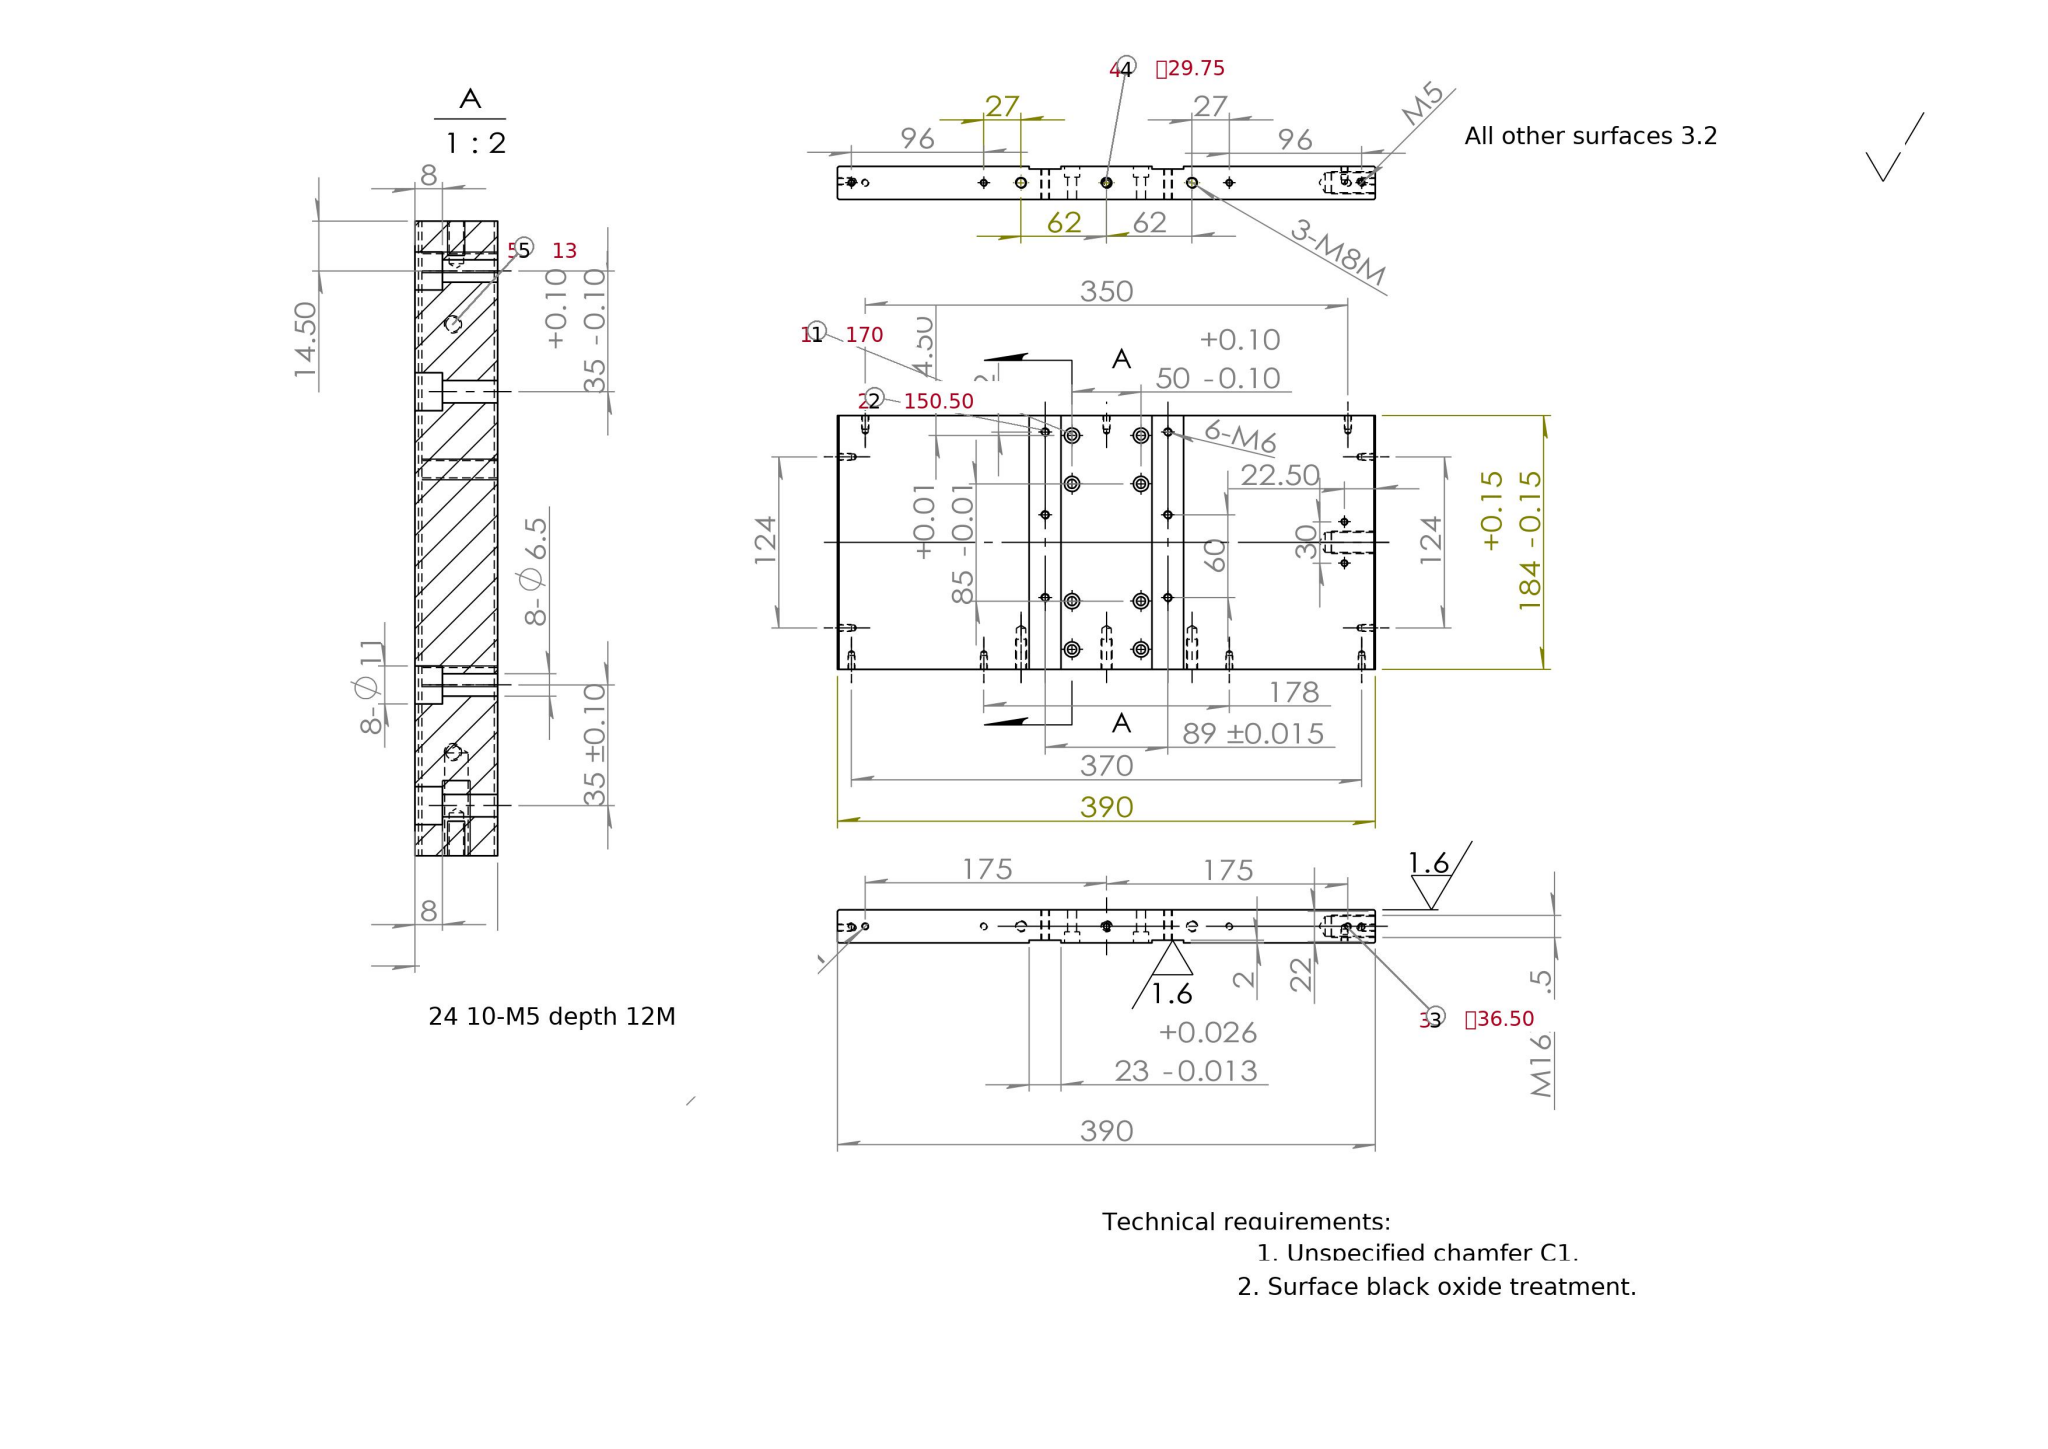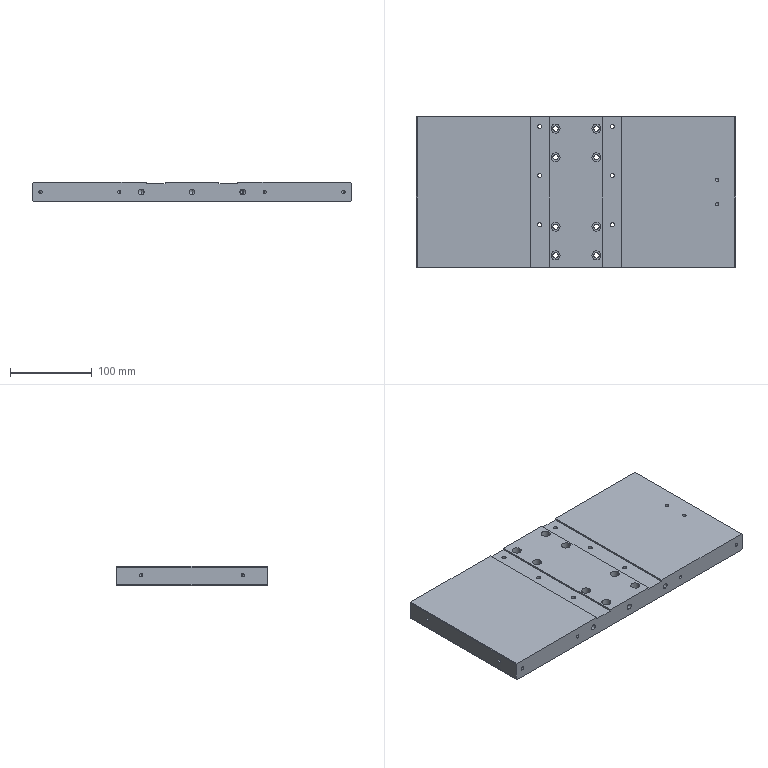Part | SolidWorks | mm | 1 solid | 138 faces | box 390 x 184 x 24 mm | volume 1680131 mm3 | cylinder 78 | cone 34 | plane 26 | commonest cylinder face diameters 4.2 x26 11 x16 6.5 x16 5 x12 6.8 x6 14.5 x2
build123d program:
from build123d import *

# Parameters (mm, degrees)
SKETCH1_W                            = 390
SKETCH1_H                            = 184
EXTRUDE1_DEPTH                       = 24
SKETCH2_R                            = 3.25
EXTRUDE2_DEPTH                       = 24
SKETCH3_R                            = 5.5
EXTRUDE3_DEPTH                       = 8
M5_TAPPED_HOLE2_AT_2_COUNT           = 2
M5_TAPPED_HOLE2_AT_2_PITCH           = 27.073
LPATTERN2_COUNT                      = 3
LPATTERN2_PITCH                      = 175
M5_TAPPED_HOLE5_D                    = 4.2
M5_TAPPED_HOLE5_DEPTH                = 12.4
M5_TAPPED_HOLE5_TIP                  = 1.262
M5_TAPPED_HOLE6_D                    = 4.2
M5_TAPPED_HOLE6_DEPTH                = 12.4
M5_TAPPED_HOLE6_TIP                  = 1.262
M16X1_5_TAPPED_HOLE1_D               = 14.5
M16X1_5_TAPPED_HOLE1_DEPTH           = 36.5
M16X1_5_TAPPED_HOLE1_TIP             = 4.356
M16X1_5_TAPPED_HOLE1_ON_FACE_2_D     = 14.5
M16X1_5_TAPPED_HOLE1_ON_FACE_2_DEPTH = 36.5
M16X1_5_TAPPED_HOLE1_ON_FACE_2_TIP   = 4.356
SKETCH27_W                           = 23
SKETCH27_H                           = 184
EXTRUDE4_DEPTH                       = 2
M6_TAPPED_HOLE1_D                    = 5
LPATTERN3_COUNT                      = 2
LPATTERN3_PITCH                      = 89
M8_TAPPED_HOLE1_D                    = 6.8
M8_TAPPED_HOLE1_DEPTH                = 29.75
M8_TAPPED_HOLE1_TIP                  = 2.043
M5_TAPPED_HOLE7_D                    = 4.2
M5_TAPPED_HOLE7_DEPTH                = 12.4
M5_TAPPED_HOLE7_TIP                  = 1.262
M5_TAPPED_HOLE8_D                    = 4.2
M5_TAPPED_HOLE8_DEPTH                = 12.4
M5_TAPPED_HOLE8_TIP                  = 1.262
CHAMFER1_SIZE                        = 1


with BuildPart() as part:
    # Sketch1 → Extrude1 (new body)
    with BuildSketch(Plane.XY):
        with Locations((195, 92)):
            Rectangle(SKETCH1_W, SKETCH1_H)
    extrude(amount=EXTRUDE1_DEPTH)

    # Sketch2 → Extrude2 (cut)
    with BuildSketch(Plane.XY.offset(24)):
        with Locations((170, 169.5)):
            Circle(SKETCH2_R)
        with Locations(Location((220, 169.5, 0), (0, 0, 180))):
            Circle(SKETCH2_R)
        with Locations((220, 134.5)):
            Circle(SKETCH2_R)
        with Locations(Location((170, 134.5, 0), (0, 0, 180))):
            Circle(SKETCH2_R)
        with Locations((170, 49.5)):
            Circle(SKETCH2_R)
        with Locations(Location((220, 49.5, 0), (0, 0, 180))):
            Circle(SKETCH2_R)
        with Locations((220, 14.5)):
            Circle(SKETCH2_R)
        with Locations(Location((170, 14.5, 0), (0, 0, 180))):
            Circle(SKETCH2_R)
    extrude(amount=-EXTRUDE2_DEPTH, mode=Mode.SUBTRACT)

    # Sketch3 → Extrude3 (cut)
    with BuildSketch(Plane.XY.offset(24)):
        with Locations((170, 169.5)):
            Circle(SKETCH3_R)
        with Locations(Location((220, 169.5, 0), (0, 0, 180))):
            Circle(SKETCH3_R)
        with Locations((220, 134.5)):
            Circle(SKETCH3_R)
        with Locations(Location((170, 134.5, 0), (0, 0, 180))):
            Circle(SKETCH3_R)
        with Locations((170, 49.5)):
            Circle(SKETCH3_R)
        with Locations(Location((220, 49.5, 0), (0, 0, 180))):
            Circle(SKETCH3_R)
        with Locations((220, 14.5)):
            Circle(SKETCH3_R)
        with Locations(Location((170, 14.5, 0), (0, 0, 180))):
            Circle(SKETCH3_R)
    extrude(amount=-EXTRUDE3_DEPTH, mode=Mode.SUBTRACT)

    # Sketch16 → M5 Tapped Hole2 (revolve, cut)
    with BuildSketch(Plane(origin=(20, 184, 12), x_dir=(0, 0, 1), z_dir=(1, 0, 0))):
        Polygon((0, 0), (0, 13.662), (2.1, 12.4), (2.1, 0), align=None)
    m5_tapped_hole2 = revolve(axis=Axis((20, 190.35, 12), (0, -1, 0)), mode=Mode.SUBTRACT)

    # M5 Tapped Hole2 at 2: M5 Tapped Hole2 ×2
    with Locations(*[Vector(-0.3525, 0, 0.9358) * (i * M5_TAPPED_HOLE2_AT_2_PITCH) for i in range(1, M5_TAPPED_HOLE2_AT_2_COUNT)]):
        add(m5_tapped_hole2, mode=Mode.SUBTRACT)

    # LPattern2: M5 Tapped Hole2 ×3
    with Locations(*[(i * LPATTERN2_PITCH, 0, 0) for i in range(1, LPATTERN2_COUNT)]):
        add(m5_tapped_hole2, mode=Mode.SUBTRACT)

    # LPattern2 copy 1 sketch → LPattern2 copy 1 (revolve, cut)
    with BuildSketch(Plane(origin=(185.456, 184, 37.335), x_dir=(0, 0, 1), z_dir=(1, 0, 0))):
        Polygon((0, 0), (0, 13.662), (2.1, 12.4), (2.1, 0), align=None)
    revolve(axis=Axis((185.456, 190.35, 37.335), (0, -1, 0)), mode=Mode.SUBTRACT)

    # LPattern2 copy 2 sketch → LPattern2 copy 2 (revolve, cut)
    with BuildSketch(Plane(origin=(360.456, 184, 37.335), x_dir=(0, 0, 1), z_dir=(1, 0, 0))):
        Polygon((0, 0), (0, 13.662), (2.1, 12.4), (2.1, 0), align=None)
    revolve(axis=Axis((360.456, 190.35, 37.335), (0, -1, 0)), mode=Mode.SUBTRACT)

    # M5 Tapped Hole5
    with Locations(Plane(origin=(390, 154, 13), x_dir=(0, 0, 1), z_dir=(1, 0, 0))):
        with Locations((0, 0), (0, 124)):
            Hole(M5_TAPPED_HOLE5_D / 2, depth=M5_TAPPED_HOLE5_DEPTH)
            with Locations((0, 0, -(M5_TAPPED_HOLE5_DEPTH + M5_TAPPED_HOLE5_TIP / 2))):  # 118° drill point
                Cone(0, M5_TAPPED_HOLE5_D / 2, M5_TAPPED_HOLE5_TIP, mode=Mode.SUBTRACT)

    # M5 Tapped Hole6
    with Locations(Plane(origin=(0, 154, 13), x_dir=(0, 0, -1), z_dir=(-1, 0, 0))):
        with Locations((0, 0), (0, 124)):
            Hole(M5_TAPPED_HOLE6_D / 2, depth=M5_TAPPED_HOLE6_DEPTH)
            with Locations((0, 0, -(M5_TAPPED_HOLE6_DEPTH + M5_TAPPED_HOLE6_TIP / 2))):  # 118° drill point
                Cone(0, M5_TAPPED_HOLE6_D / 2, M5_TAPPED_HOLE6_TIP, mode=Mode.SUBTRACT)

    # M16x1.5 Tapped Hole1
    with Locations(Plane(origin=(390, 92, 12), x_dir=(0, 0, 1), z_dir=(1, 0, 0))):
        with Locations((0, 0)):
            Hole(M16X1_5_TAPPED_HOLE1_D / 2, depth=M16X1_5_TAPPED_HOLE1_DEPTH)
            with Locations((0, 0, -(M16X1_5_TAPPED_HOLE1_DEPTH + M16X1_5_TAPPED_HOLE1_TIP / 2))):  # 118° drill point
                Cone(0, M16X1_5_TAPPED_HOLE1_D / 2, M16X1_5_TAPPED_HOLE1_TIP, mode=Mode.SUBTRACT)

    # M16x1.5 Tapped Hole1 on face 2
    with Locations(Plane(origin=(0, 159.463, -37.65), x_dir=(0, 0, 1), z_dir=(1, 0, 0))):
        with Locations((0, 0)):
            Hole(M16X1_5_TAPPED_HOLE1_ON_FACE_2_D / 2, depth=M16X1_5_TAPPED_HOLE1_ON_FACE_2_DEPTH)
            with Locations((0, 0, -(M16X1_5_TAPPED_HOLE1_ON_FACE_2_DEPTH + M16X1_5_TAPPED_HOLE1_ON_FACE_2_TIP / 2))):  # 118° drill point
                Cone(0, M16X1_5_TAPPED_HOLE1_ON_FACE_2_D / 2, M16X1_5_TAPPED_HOLE1_ON_FACE_2_TIP, mode=Mode.SUBTRACT)

    # Sketch27 → Extrude4 (cut)
    with BuildSketch(Plane.XY.offset(24)):
        with Locations((239.5, 92)):
            Rectangle(SKETCH27_W, SKETCH27_H)
        with Locations((150.5, 92)):
            Rectangle(SKETCH27_W, SKETCH27_H)
    extrude(amount=-EXTRUDE4_DEPTH, mode=Mode.SUBTRACT)

    # M6 Tapped Hole1 (through all)
    with Locations(Plane(origin=(150.5, 172, 22), x_dir=(1, 0, 0), z_dir=(0, 0, 1))):
        with Locations((0, 0), (0, -60), (0, -120)):
            m6_tapped_hole1 = Hole(M6_TAPPED_HOLE1_D / 2)

    # LPattern3: M6 Tapped Hole1 ×2
    with Locations(*[(i * LPATTERN3_PITCH, 0, 0) for i in range(1, LPATTERN3_COUNT)]):
        add(m6_tapped_hole1, mode=Mode.SUBTRACT)

    # M8 Tapped Hole1
    with Locations(Plane(origin=(195, 0, 12), x_dir=(0, 0, -1), z_dir=(0, -1, 0))):
        with Locations((0, 0), (0, -62), (0, 62)):
            Hole(M8_TAPPED_HOLE1_D / 2, depth=M8_TAPPED_HOLE1_DEPTH)
            with Locations((0, 0, -(M8_TAPPED_HOLE1_DEPTH + M8_TAPPED_HOLE1_TIP / 2))):  # 118° drill point
                Cone(0, M8_TAPPED_HOLE1_D / 2, M8_TAPPED_HOLE1_TIP, mode=Mode.SUBTRACT)

    # M5 Tapped Hole7
    with Locations(Plane(origin=(10, 0, 12), x_dir=(0, 0, -1), z_dir=(0, -1, 0))):
        with Locations((0, 0), (0, 96), (0, 274), (0, 370)):
            Hole(M5_TAPPED_HOLE7_D / 2, depth=M5_TAPPED_HOLE7_DEPTH)
            with Locations((0, 0, -(M5_TAPPED_HOLE7_DEPTH + M5_TAPPED_HOLE7_TIP / 2))):  # 118° drill point
                Cone(0, M5_TAPPED_HOLE7_D / 2, M5_TAPPED_HOLE7_TIP, mode=Mode.SUBTRACT)

    # M5 Tapped Hole8
    with Locations(Plane.XY.offset(24)):
        with Locations((367.5, 107), (367.5, 77)):
            Hole(M5_TAPPED_HOLE8_D / 2, depth=M5_TAPPED_HOLE8_DEPTH)
            with Locations((0, 0, -(M5_TAPPED_HOLE8_DEPTH + M5_TAPPED_HOLE8_TIP / 2))):  # 118° drill point
                Cone(0, M5_TAPPED_HOLE8_D / 2, M5_TAPPED_HOLE8_TIP, mode=Mode.SUBTRACT)

    # Chamfer1
    chamfer1_edges = [part.edges().sort_by_distance(p)[0] for p in [
        (390, 92, 24),
        (0, 92, 24),
        (390, 92, 0),
        (0, 92, 0),
    ]]
    chamfer(chamfer1_edges, length=CHAMFER1_SIZE)


solid = part.part